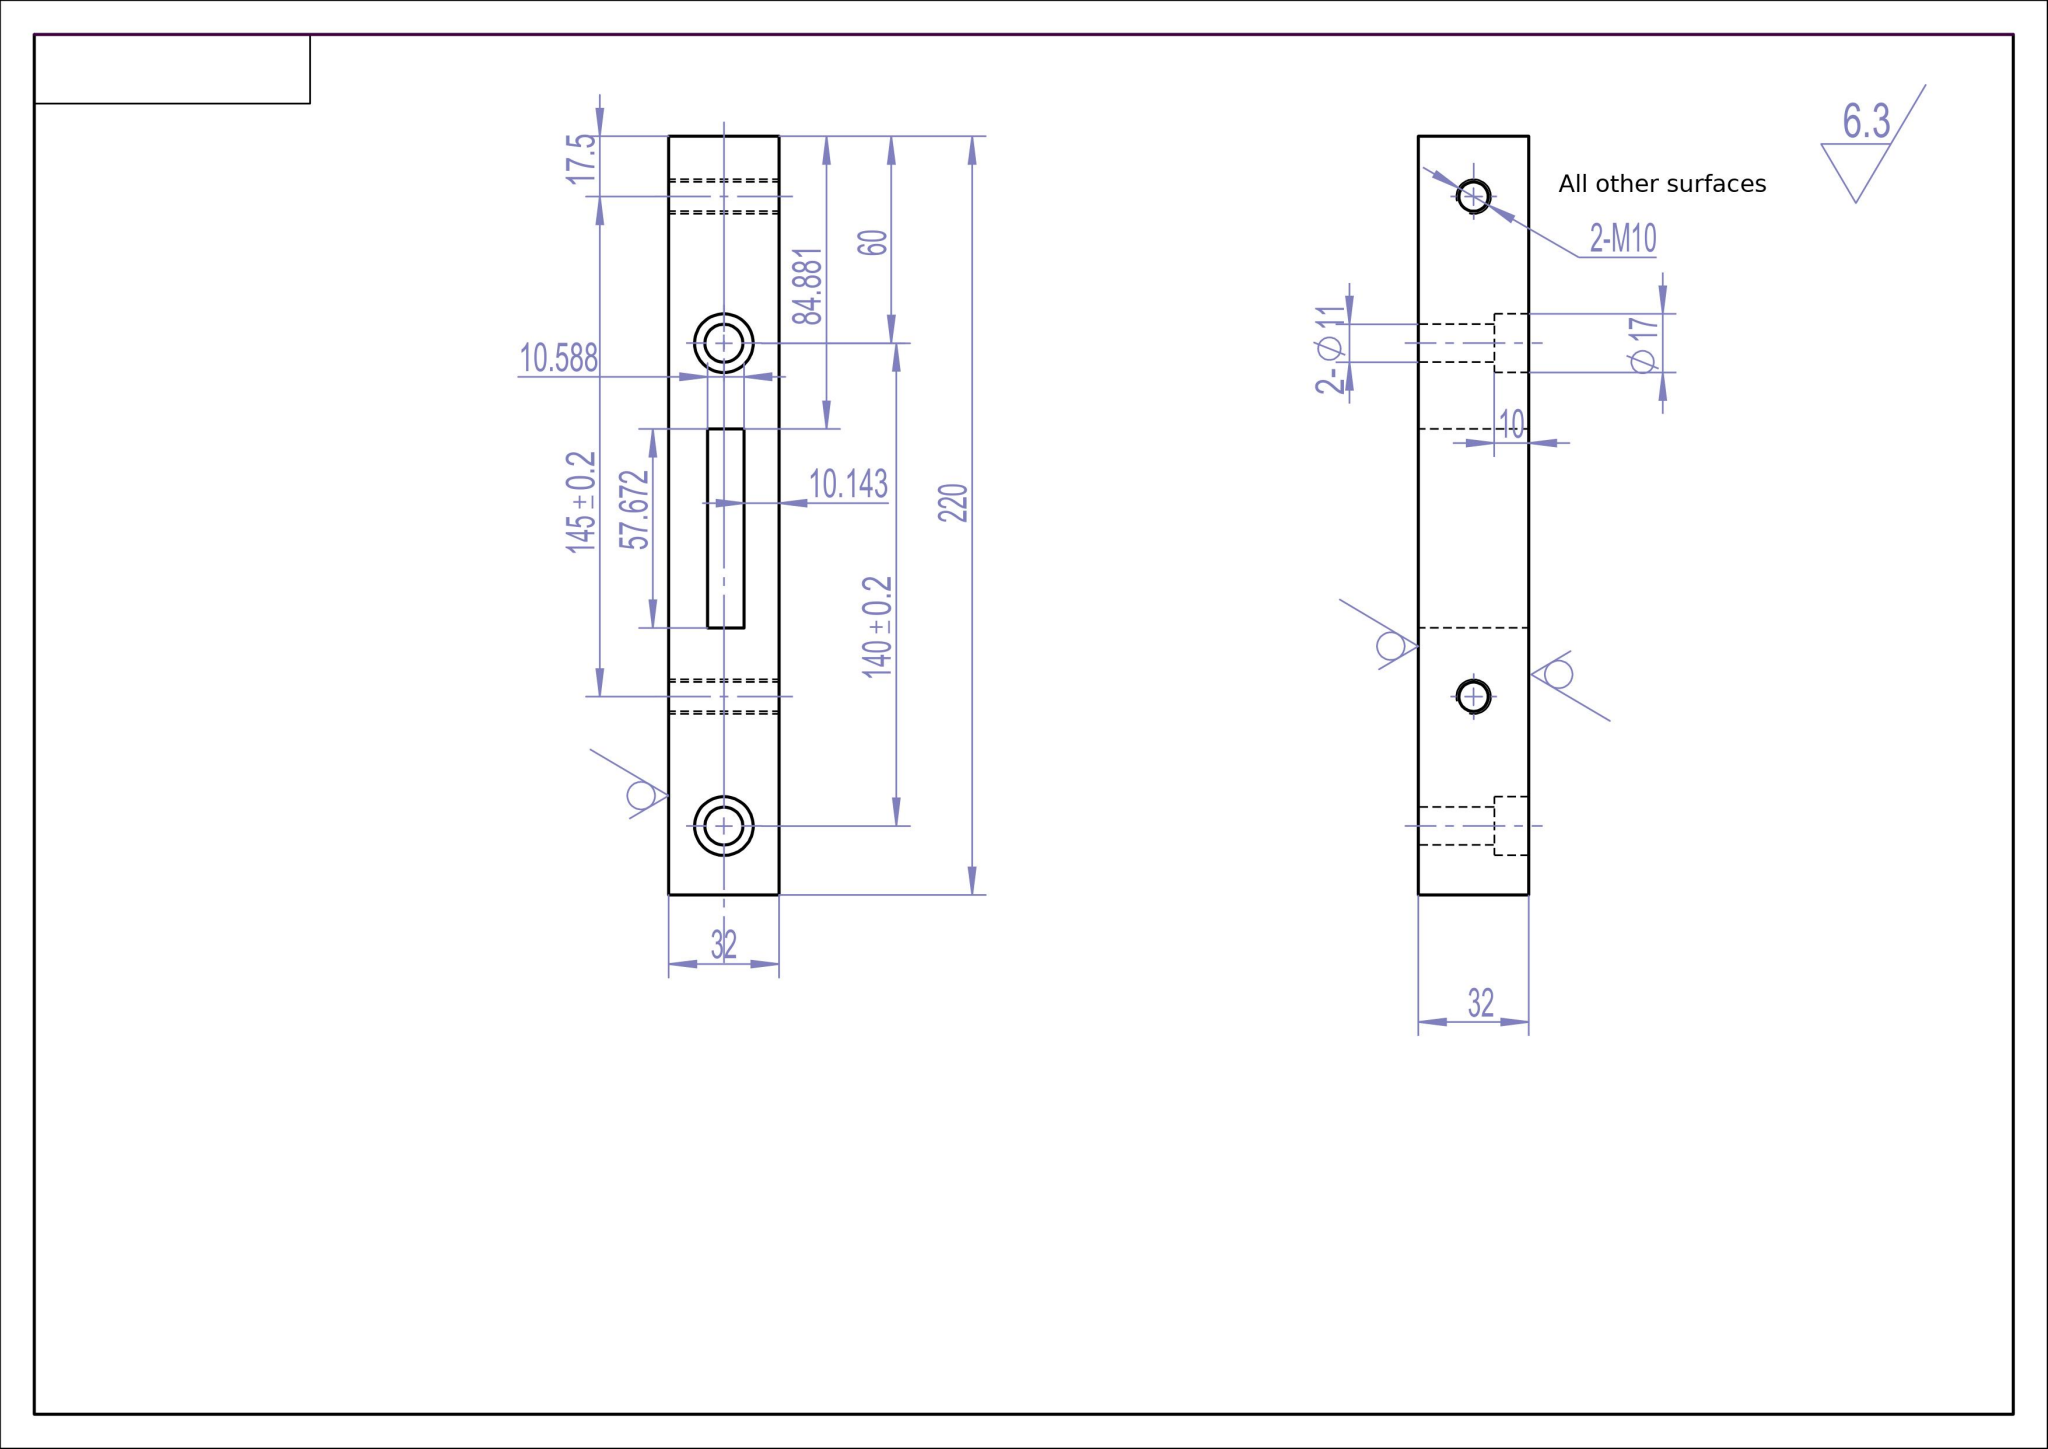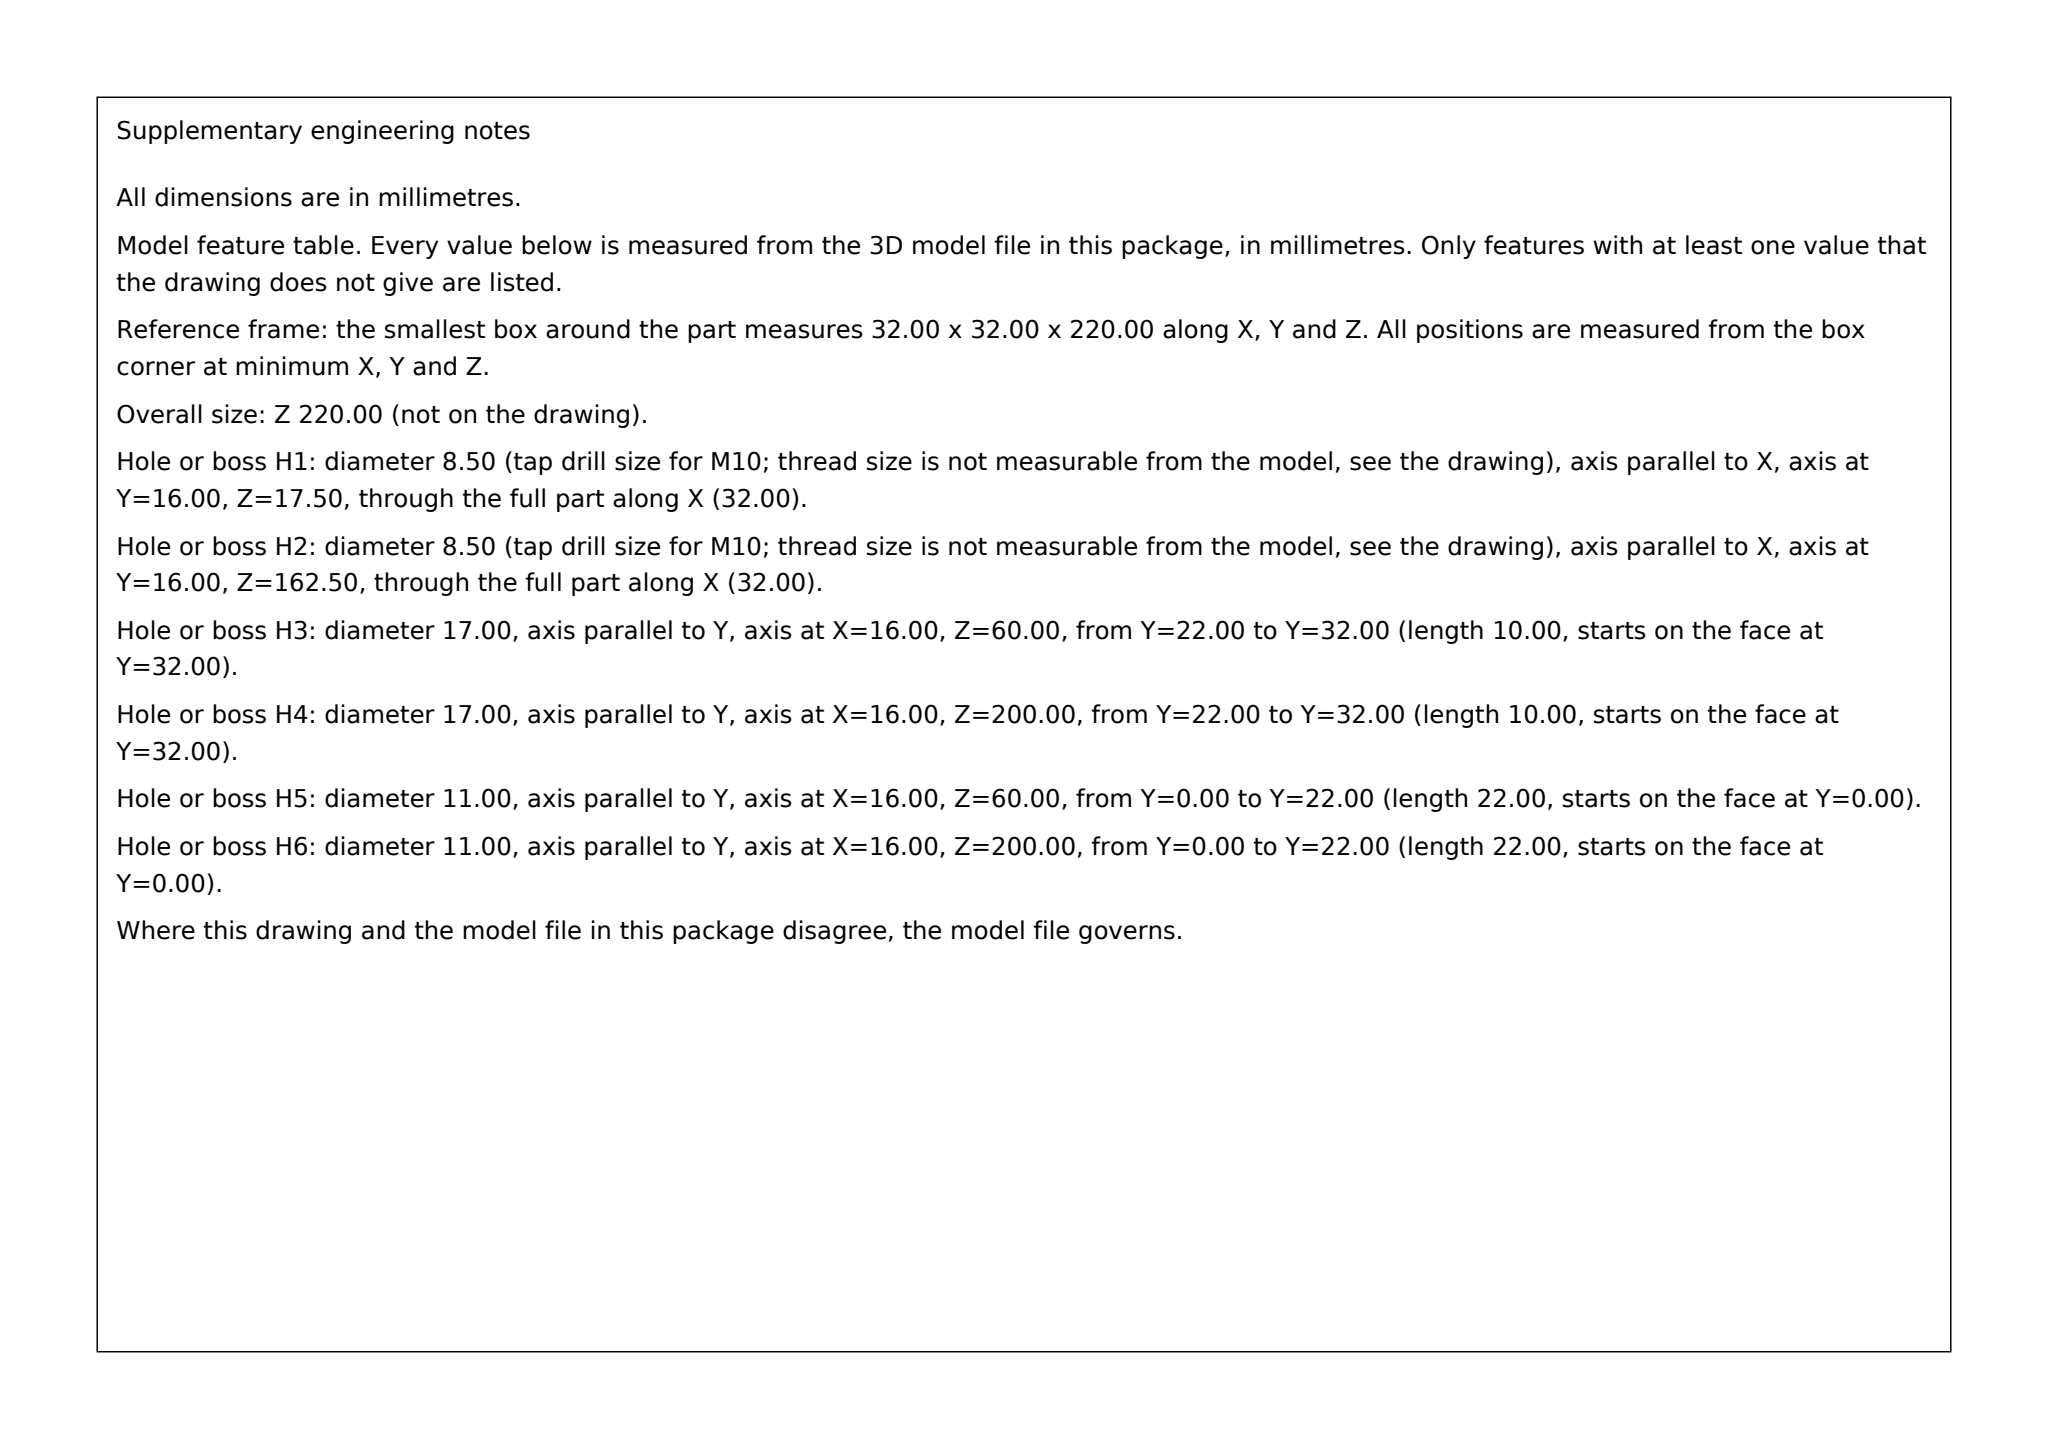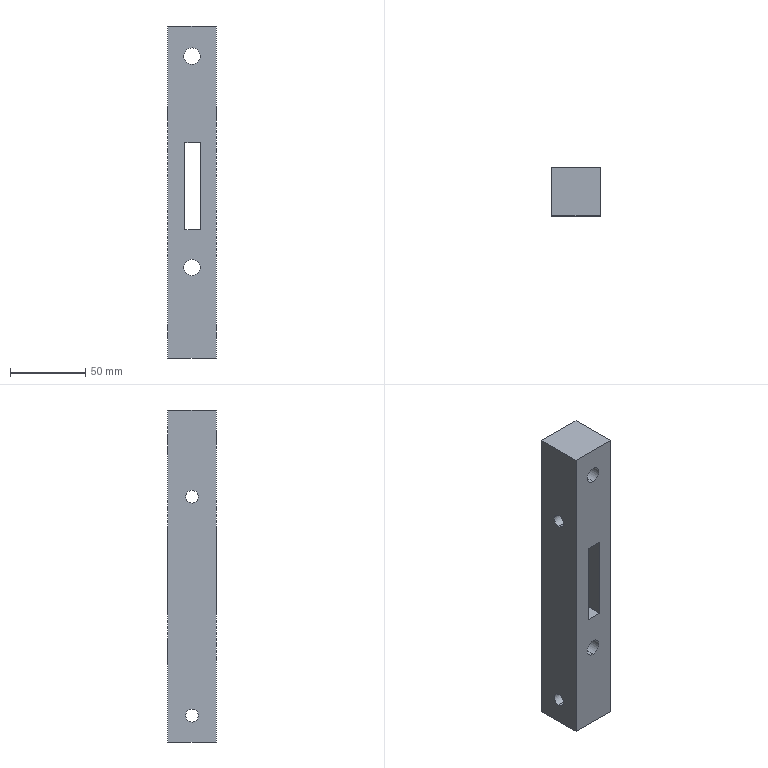Part | SolidWorks | mm | 1 solid | 24 faces | box 32 x 32 x 220 mm | volume 193387 mm3 | cylinder 12 | plane 12 | commonest cylinder face diameters 8.5 x4 11 x4 17 x4
build123d program:
from build123d import *

# Parameters (mm, degrees)
SKETCH1_W              = 32
SKETCH1_H              = 32
BOSS_EXTRUDE1_DEPTH    = 110
SKETCH2_R              = 8.5
CUT_EXTRUDE1_DEPTH     = 10
SKETCH3_R              = 5.5
CUT_EXTRUDE2_DEPTH     = 30
M10_TAPPED_HOLE1_D     = 8.5
M10_TAPPED_HOLE1_DEPTH = 44.5
M10_TAPPED_HOLE1_TIP   = 2.554
SKETCH6_W              = 10.588
SKETCH6_H              = 57.672
CUT_EXTRUDE3_DEPTH     = 95


with BuildPart() as part:
    # Sketch1 → Boss-Extrude1 (new, symmetric)
    with BuildSketch(Plane.XY):
        with Locations((-8.754, 3.057)):
            Rectangle(SKETCH1_W, SKETCH1_H)
    extrude(amount=BOSS_EXTRUDE1_DEPTH, both=True)

    # Sketch2 → Cut-Extrude1 (cut)
    with BuildSketch(Plane(origin=(0, 19.057, 0), x_dir=(1, 0, 0), z_dir=(0, 1, 0))):
        with Locations(Location((-8.754, 50, 0), (0, 0, 270))):
            Circle(SKETCH2_R)
        with Locations(Location((-8.754, -90, 0), (0, 0, 270))):
            Circle(SKETCH2_R)
    extrude(amount=-CUT_EXTRUDE1_DEPTH, mode=Mode.SUBTRACT)

    # Sketch3 → Cut-Extrude2 (cut)
    with BuildSketch(Plane(origin=(0, 9.057, 0), x_dir=(1, 0, 0), z_dir=(0, 1, 0))):
        with Locations(Location((-8.754, 50, 0), (0, 0, 270))):
            Circle(SKETCH3_R)
        with Locations(Location((-8.754, -90, 0), (0, 0, 270))):
            Circle(SKETCH3_R)
    extrude(amount=-CUT_EXTRUDE2_DEPTH, mode=Mode.SUBTRACT)

    # M10 Tapped Hole1
    with Locations(Plane(origin=(-24.754, 3.057, -92.5), x_dir=(0, -1, 0), z_dir=(-1, 0, 0))):
        with Locations((0, 0), (0, 145)):
            Hole(M10_TAPPED_HOLE1_D / 2, depth=M10_TAPPED_HOLE1_DEPTH)
            with Locations((0, 0, -(M10_TAPPED_HOLE1_DEPTH + M10_TAPPED_HOLE1_TIP / 2))):  # 118° drill point
                Cone(0, M10_TAPPED_HOLE1_D / 2, M10_TAPPED_HOLE1_TIP, mode=Mode.SUBTRACT)

    # Sketch6 → Cut-Extrude3 (cut)
    with BuildSketch(Plane(origin=(0, 19.057, 0), x_dir=(1, 0, 0), z_dir=(0, 1, 0))):
        with Locations((-8.191, -3.717)):
            Rectangle(SKETCH6_W, SKETCH6_H)
    extrude(amount=-CUT_EXTRUDE3_DEPTH, mode=Mode.SUBTRACT)


solid = part.part